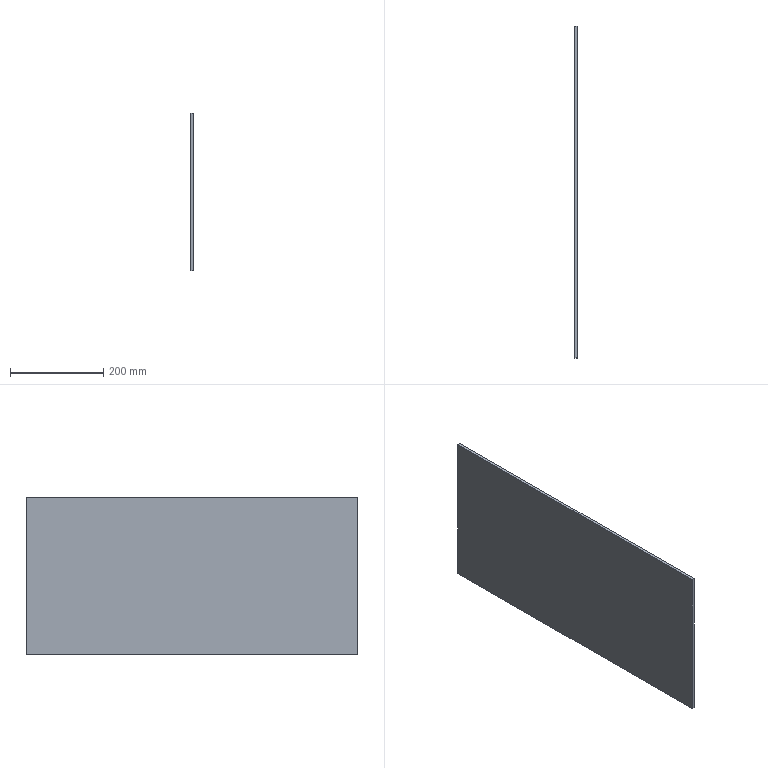Component | SolidWorks | RibPlate-16 | 1 solid | 6 faces | box 6 x 710 x 338 mm | volume 1439880 mm3 | plane 6 | material Plain Carbon Steel
STEP:
#1=COLOUR_RGB('',0.7922,0.8196,0.9333);
#2=FILL_AREA_STYLE_COLOUR('',#1);
#3=FILL_AREA_STYLE('',(#2));
#4=SURFACE_STYLE_FILL_AREA(#3);
#5=SURFACE_SIDE_STYLE('',(#4));
#6=SURFACE_STYLE_USAGE(.BOTH.,#5);
#7=PRESENTATION_STYLE_ASSIGNMENT((#6));
#8=CARTESIAN_POINT('',(167.596,126.37,154.106));
#9=VERTEX_POINT('',#8);
#10=CARTESIAN_POINT('',(167.596,126.37,140.799));
#11=VERTEX_POINT('',#10);
#12=CARTESIAN_POINT('',(167.596,126.37,140.799));
#13=DIRECTION('',(0.,0.,-1.));
#14=VECTOR('',#13,39.37);
#15=LINE('',#12,#14);
#16=EDGE_CURVE('',#9,#11,#15,.T.);
#17=ORIENTED_EDGE('',*,*,#16,.F.);
#18=CARTESIAN_POINT('',(167.832,126.37,154.106));
#19=VERTEX_POINT('',#18);
#20=CARTESIAN_POINT('',(167.832,126.37,154.106));
#21=DIRECTION('',(-1.,-0.,0.));
#22=VECTOR('',#21,39.37);
#23=LINE('',#20,#22);
#24=EDGE_CURVE('',#19,#9,#23,.T.);
#25=ORIENTED_EDGE('',*,*,#24,.F.);
#26=CARTESIAN_POINT('',(167.832,126.37,140.799));
#27=VERTEX_POINT('',#26);
#28=CARTESIAN_POINT('',(167.832,126.37,140.799));
#29=DIRECTION('',(0.,0.,-1.));
#30=VECTOR('',#29,39.37);
#31=LINE('',#28,#30);
#32=EDGE_CURVE('',#19,#27,#31,.T.);
#33=ORIENTED_EDGE('',*,*,#32,.T.);
#34=CARTESIAN_POINT('',(167.832,126.37,140.799));
#35=DIRECTION('',(-1.,-0.,0.));
#36=VECTOR('',#35,39.37);
#37=LINE('',#34,#36);
#38=EDGE_CURVE('',#27,#11,#37,.T.);
#39=ORIENTED_EDGE('',*,*,#38,.T.);
#40=EDGE_LOOP('',(#17,#25,#33,#39));
#41=FACE_OUTER_BOUND('',#40,.T.);
#42=CARTESIAN_POINT('',(167.832,126.37,140.799));
#43=DIRECTION('',(-0.,1.,0.));
#44=DIRECTION('',(0.,0.,-1.));
#45=AXIS2_PLACEMENT_3D('',#42,#43,#44);
#46=PLANE('',#45);
#47=ADVANCED_FACE('',(#41),#46,.T.);
#48=CARTESIAN_POINT('',(167.596,98.417,154.106));
#49=VERTEX_POINT('',#48);
#50=CARTESIAN_POINT('',(167.596,98.417,154.106));
#51=DIRECTION('',(-0.,1.,0.));
#52=VECTOR('',#51,39.37);
#53=LINE('',#50,#52);
#54=EDGE_CURVE('',#49,#9,#53,.T.);
#55=ORIENTED_EDGE('',*,*,#54,.F.);
#56=CARTESIAN_POINT('',(167.832,98.417,154.106));
#57=VERTEX_POINT('',#56);
#58=CARTESIAN_POINT('',(167.832,98.417,154.106));
#59=DIRECTION('',(-1.,-0.,0.));
#60=VECTOR('',#59,39.37);
#61=LINE('',#58,#60);
#62=EDGE_CURVE('',#57,#49,#61,.T.);
#63=ORIENTED_EDGE('',*,*,#62,.F.);
#64=CARTESIAN_POINT('',(167.832,98.417,154.106));
#65=DIRECTION('',(-0.,1.,0.));
#66=VECTOR('',#65,39.37);
#67=LINE('',#64,#66);
#68=EDGE_CURVE('',#57,#19,#67,.T.);
#69=ORIENTED_EDGE('',*,*,#68,.T.);
#70=ORIENTED_EDGE('',*,*,#24,.T.);
#71=EDGE_LOOP('',(#55,#63,#69,#70));
#72=FACE_OUTER_BOUND('',#71,.T.);
#73=CARTESIAN_POINT('',(167.832,98.417,154.106));
#74=DIRECTION('',(0.,0.,1.));
#75=DIRECTION('',(-0.,1.,0.));
#76=AXIS2_PLACEMENT_3D('',#73,#74,#75);
#77=PLANE('',#76);
#78=ADVANCED_FACE('',(#72),#77,.T.);
#79=CARTESIAN_POINT('',(167.596,98.417,140.799));
#80=VERTEX_POINT('',#79);
#81=CARTESIAN_POINT('',(167.596,98.417,140.799));
#82=DIRECTION('',(-0.,0.,1.));
#83=VECTOR('',#82,39.37);
#84=LINE('',#81,#83);
#85=EDGE_CURVE('',#80,#49,#84,.T.);
#86=ORIENTED_EDGE('',*,*,#85,.F.);
#87=CARTESIAN_POINT('',(167.832,98.417,140.799));
#88=VERTEX_POINT('',#87);
#89=CARTESIAN_POINT('',(167.832,98.417,140.799));
#90=DIRECTION('',(-1.,-0.,0.));
#91=VECTOR('',#90,39.37);
#92=LINE('',#89,#91);
#93=EDGE_CURVE('',#88,#80,#92,.T.);
#94=ORIENTED_EDGE('',*,*,#93,.F.);
#95=CARTESIAN_POINT('',(167.832,98.417,140.799));
#96=DIRECTION('',(-0.,0.,1.));
#97=VECTOR('',#96,39.37);
#98=LINE('',#95,#97);
#99=EDGE_CURVE('',#88,#57,#98,.T.);
#100=ORIENTED_EDGE('',*,*,#99,.T.);
#101=ORIENTED_EDGE('',*,*,#62,.T.);
#102=EDGE_LOOP('',(#86,#94,#100,#101));
#103=FACE_OUTER_BOUND('',#102,.T.);
#104=CARTESIAN_POINT('',(167.832,98.417,140.799));
#105=DIRECTION('',(0.,-1.,0.));
#106=DIRECTION('',(-0.,0.,1.));
#107=AXIS2_PLACEMENT_3D('',#104,#105,#106);
#108=PLANE('',#107);
#109=ADVANCED_FACE('',(#103),#108,.T.);
#110=CARTESIAN_POINT('',(167.596,98.417,140.799));
#111=DIRECTION('',(0.,-1.,0.));
#112=VECTOR('',#111,39.37);
#113=LINE('',#110,#112);
#114=EDGE_CURVE('',#11,#80,#113,.T.);
#115=ORIENTED_EDGE('',*,*,#114,.F.);
#116=ORIENTED_EDGE('',*,*,#38,.F.);
#117=CARTESIAN_POINT('',(167.832,98.417,140.799));
#118=DIRECTION('',(0.,-1.,0.));
#119=VECTOR('',#118,39.37);
#120=LINE('',#117,#119);
#121=EDGE_CURVE('',#27,#88,#120,.T.);
#122=ORIENTED_EDGE('',*,*,#121,.T.);
#123=ORIENTED_EDGE('',*,*,#93,.T.);
#124=EDGE_LOOP('',(#115,#116,#122,#123));
#125=FACE_OUTER_BOUND('',#124,.T.);
#126=CARTESIAN_POINT('',(167.832,98.417,140.799));
#127=DIRECTION('',(0.,0.,-1.));
#128=DIRECTION('',(0.,-1.,0.));
#129=AXIS2_PLACEMENT_3D('',#126,#127,#128);
#130=PLANE('',#129);
#131=ADVANCED_FACE('',(#125),#130,.T.);
#132=ORIENTED_EDGE('',*,*,#32,.F.);
#133=ORIENTED_EDGE('',*,*,#68,.F.);
#134=ORIENTED_EDGE('',*,*,#99,.F.);
#135=ORIENTED_EDGE('',*,*,#121,.F.);
#136=EDGE_LOOP('',(#132,#133,#134,#135));
#137=FACE_OUTER_BOUND('',#136,.T.);
#138=CARTESIAN_POINT('',(167.832,112.394,147.452));
#139=DIRECTION('',(-1.,-0.,0.));
#140=DIRECTION('',(0.,0.,1.));
#141=AXIS2_PLACEMENT_3D('',#138,#139,#140);
#142=PLANE('',#141);
#143=ADVANCED_FACE('',(#137),#142,.F.);
#144=ORIENTED_EDGE('',*,*,#16,.T.);
#145=ORIENTED_EDGE('',*,*,#114,.T.);
#146=ORIENTED_EDGE('',*,*,#85,.T.);
#147=ORIENTED_EDGE('',*,*,#54,.T.);
#148=EDGE_LOOP('',(#144,#145,#146,#147));
#149=FACE_OUTER_BOUND('',#148,.T.);
#150=CARTESIAN_POINT('',(167.596,112.394,147.452));
#151=DIRECTION('',(-1.,-0.,0.));
#152=DIRECTION('',(0.,0.,1.));
#153=AXIS2_PLACEMENT_3D('',#150,#151,#152);
#154=PLANE('',#153);
#155=ADVANCED_FACE('',(#149),#154,.T.);
#156=CLOSED_SHELL('',(#47,#78,#109,#131,#143,#155));
#157=MANIFOLD_SOLID_BREP('',#156);
#158=STYLED_ITEM('',(#7),#157);
#159=PRESENTATION_LAYER_ASSIGNMENT('','',(#158));
#160=CARTESIAN_POINT('',(0.,0.,0.));
#161=DIRECTION('',(0.,0.,1.));
#162=DIRECTION('',(1.,0.,0.));
#163=AXIS2_PLACEMENT_3D('',#160,#161,#162);
#164=(LENGTH_UNIT()NAMED_UNIT(*)SI_UNIT($,.METRE.));
#165=LENGTH_MEASURE_WITH_UNIT(LENGTH_MEASURE(0.0254),#164);
#166=DIMENSIONAL_EXPONENTS(1.,0.,0.,0.,0.,0.,0.);
#167=(CONVERSION_BASED_UNIT('',#165)LENGTH_UNIT()NAMED_UNIT(#166));
#168=UNCERTAINTY_MEASURE_WITH_UNIT(LENGTH_MEASURE(0.00001),#167,'','');
#169=(NAMED_UNIT(*)PLANE_ANGLE_UNIT()SI_UNIT($,.RADIAN.));
#170=(NAMED_UNIT(*)SI_UNIT($,.STERADIAN.)SOLID_ANGLE_UNIT());
#171=(GEOMETRIC_REPRESENTATION_CONTEXT(3)GLOBAL_UNCERTAINTY_ASSIGNED_CONTEXT((#168))GLOBAL_UNIT_ASSIGNED_CONTEXT((#167,#169,#170))REPRESENTATION_CONTEXT('',''));
#172=ADVANCED_BREP_SHAPE_REPRESENTATION('',(#157,#163),#171);
#173=(LENGTH_UNIT()NAMED_UNIT(*)SI_UNIT($,.METRE.));
#174=LENGTH_MEASURE_WITH_UNIT(LENGTH_MEASURE(0.0254),#173);
#175=DIMENSIONAL_EXPONENTS(1.,0.,0.,0.,0.,0.,0.);
#176=(CONVERSION_BASED_UNIT('',#174)LENGTH_UNIT()NAMED_UNIT(#175));
#177=UNCERTAINTY_MEASURE_WITH_UNIT(LENGTH_MEASURE(0.00001),#176,'','');
#178=(NAMED_UNIT(*)PLANE_ANGLE_UNIT()SI_UNIT($,.RADIAN.));
#179=(NAMED_UNIT(*)SI_UNIT($,.STERADIAN.)SOLID_ANGLE_UNIT());
#180=(GEOMETRIC_REPRESENTATION_CONTEXT(3)GLOBAL_UNCERTAINTY_ASSIGNED_CONTEXT((#177))GLOBAL_UNIT_ASSIGNED_CONTEXT((#176,#178,#179))REPRESENTATION_CONTEXT('',''));
#181=MECHANICAL_DESIGN_GEOMETRIC_PRESENTATION_REPRESENTATION('',(#158),#180);